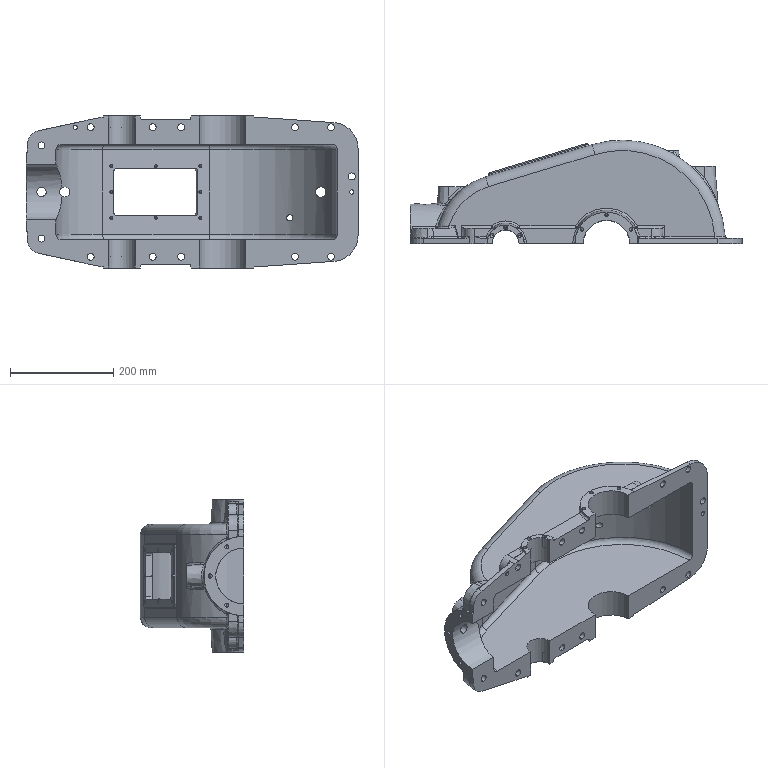Component | SolidWorks | MachineCover-1 | 1 solid | 368 faces | volume 3665897 mm3 | cylinder 154 | plane 77 | cone 49 | spline 40 | torus 30 | sphere 18 | commonest cylinder face diameters 8 x51 13.5 x26 6 x20 10 x13 6.8 x12 20 x6 44 x4 18 x2